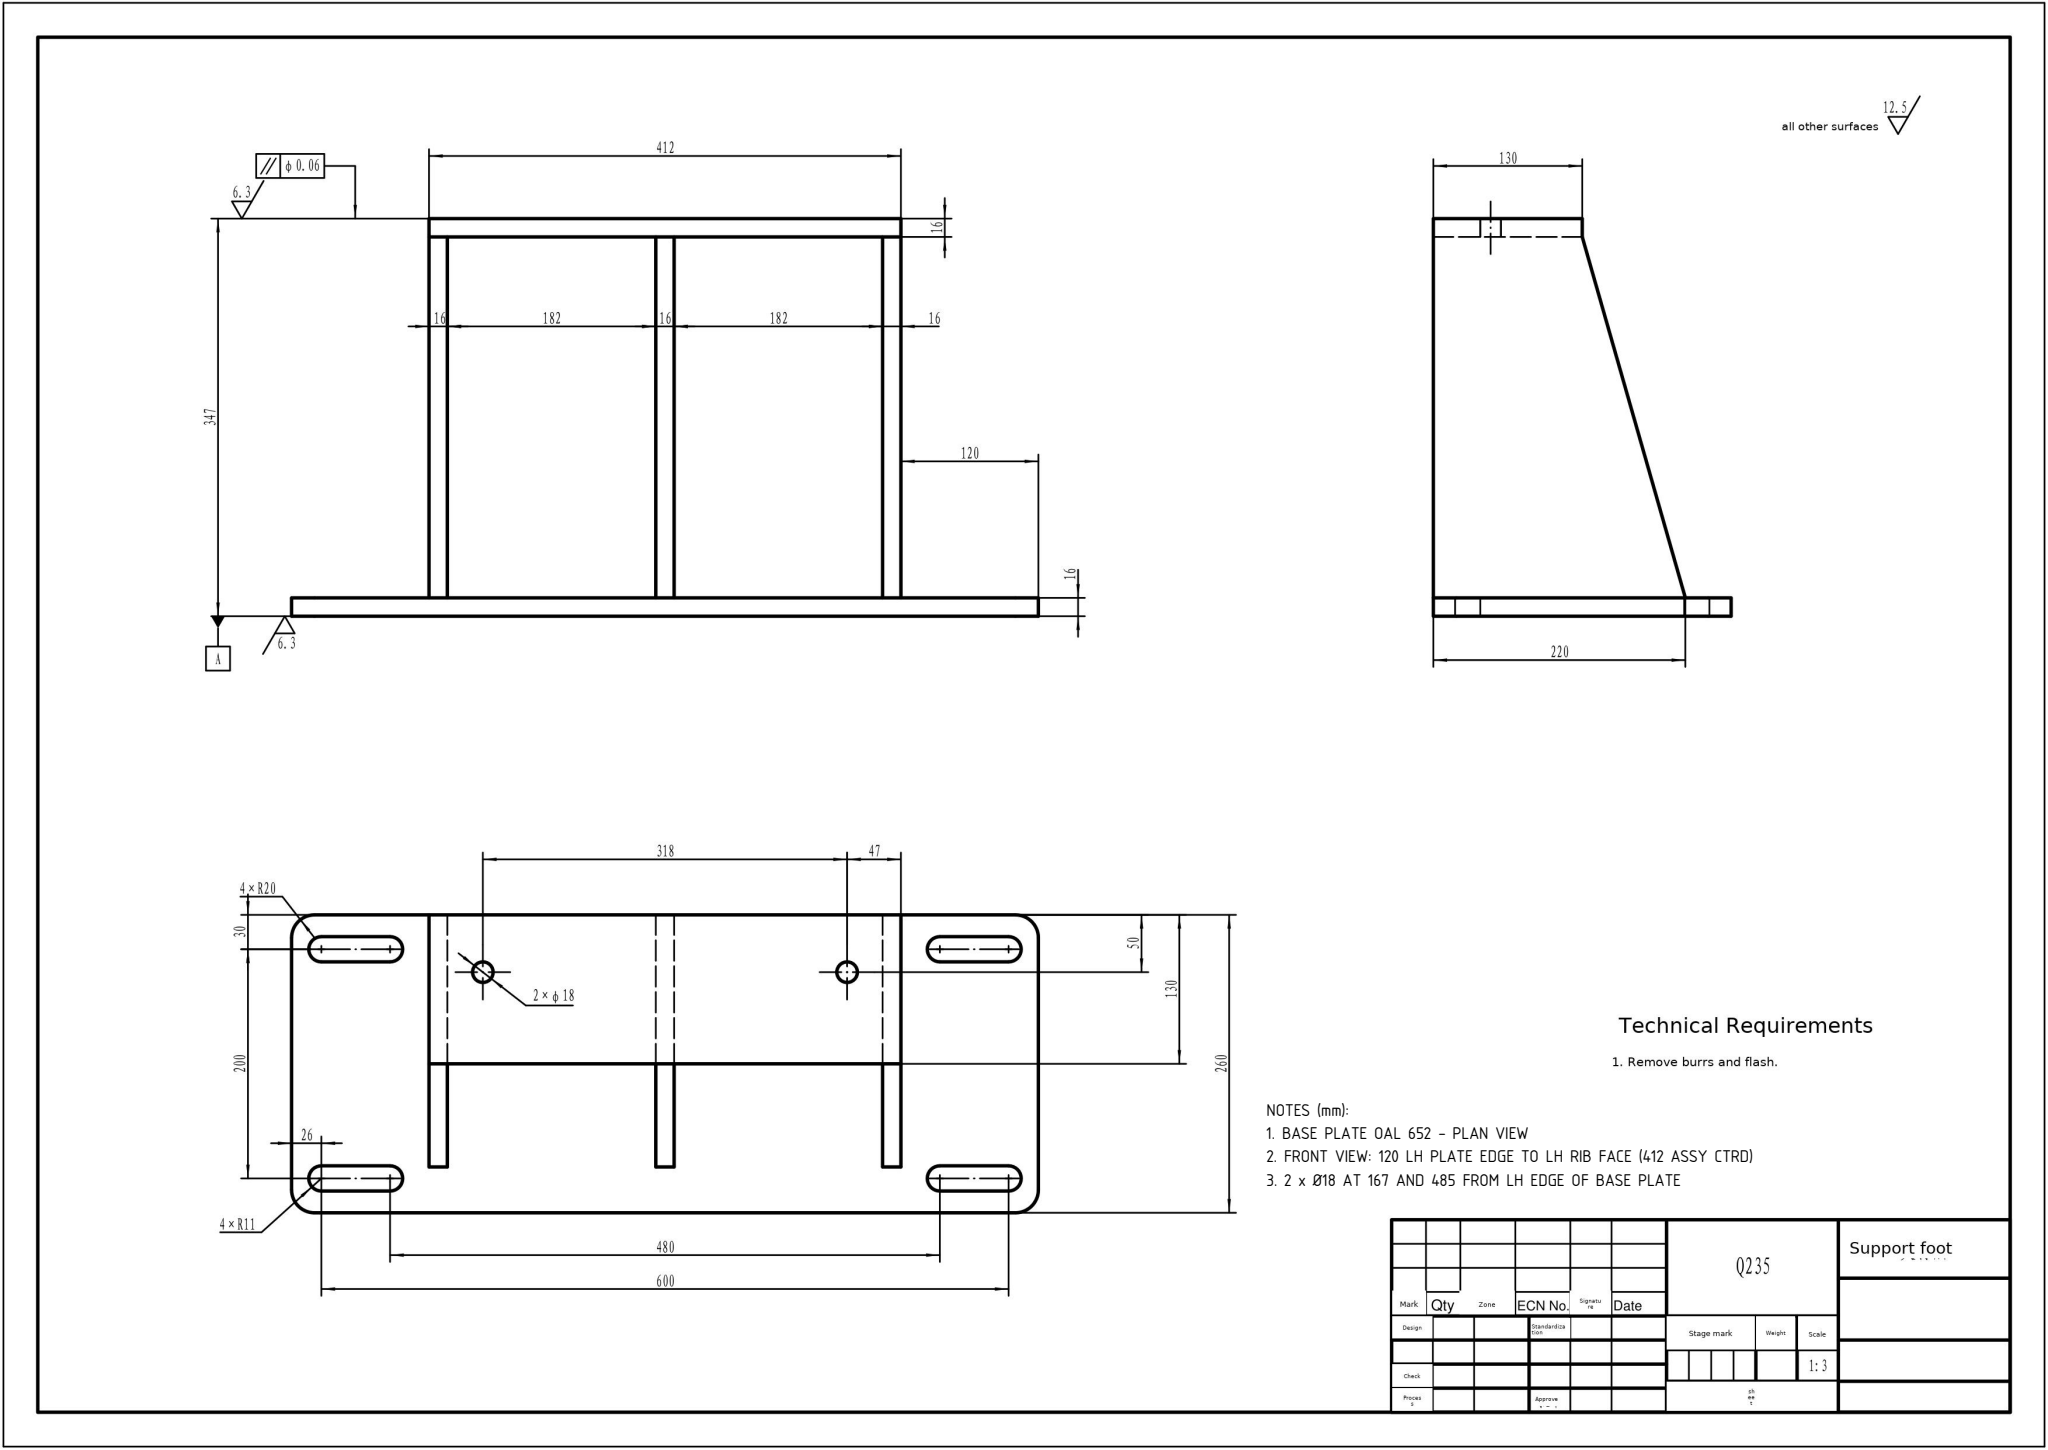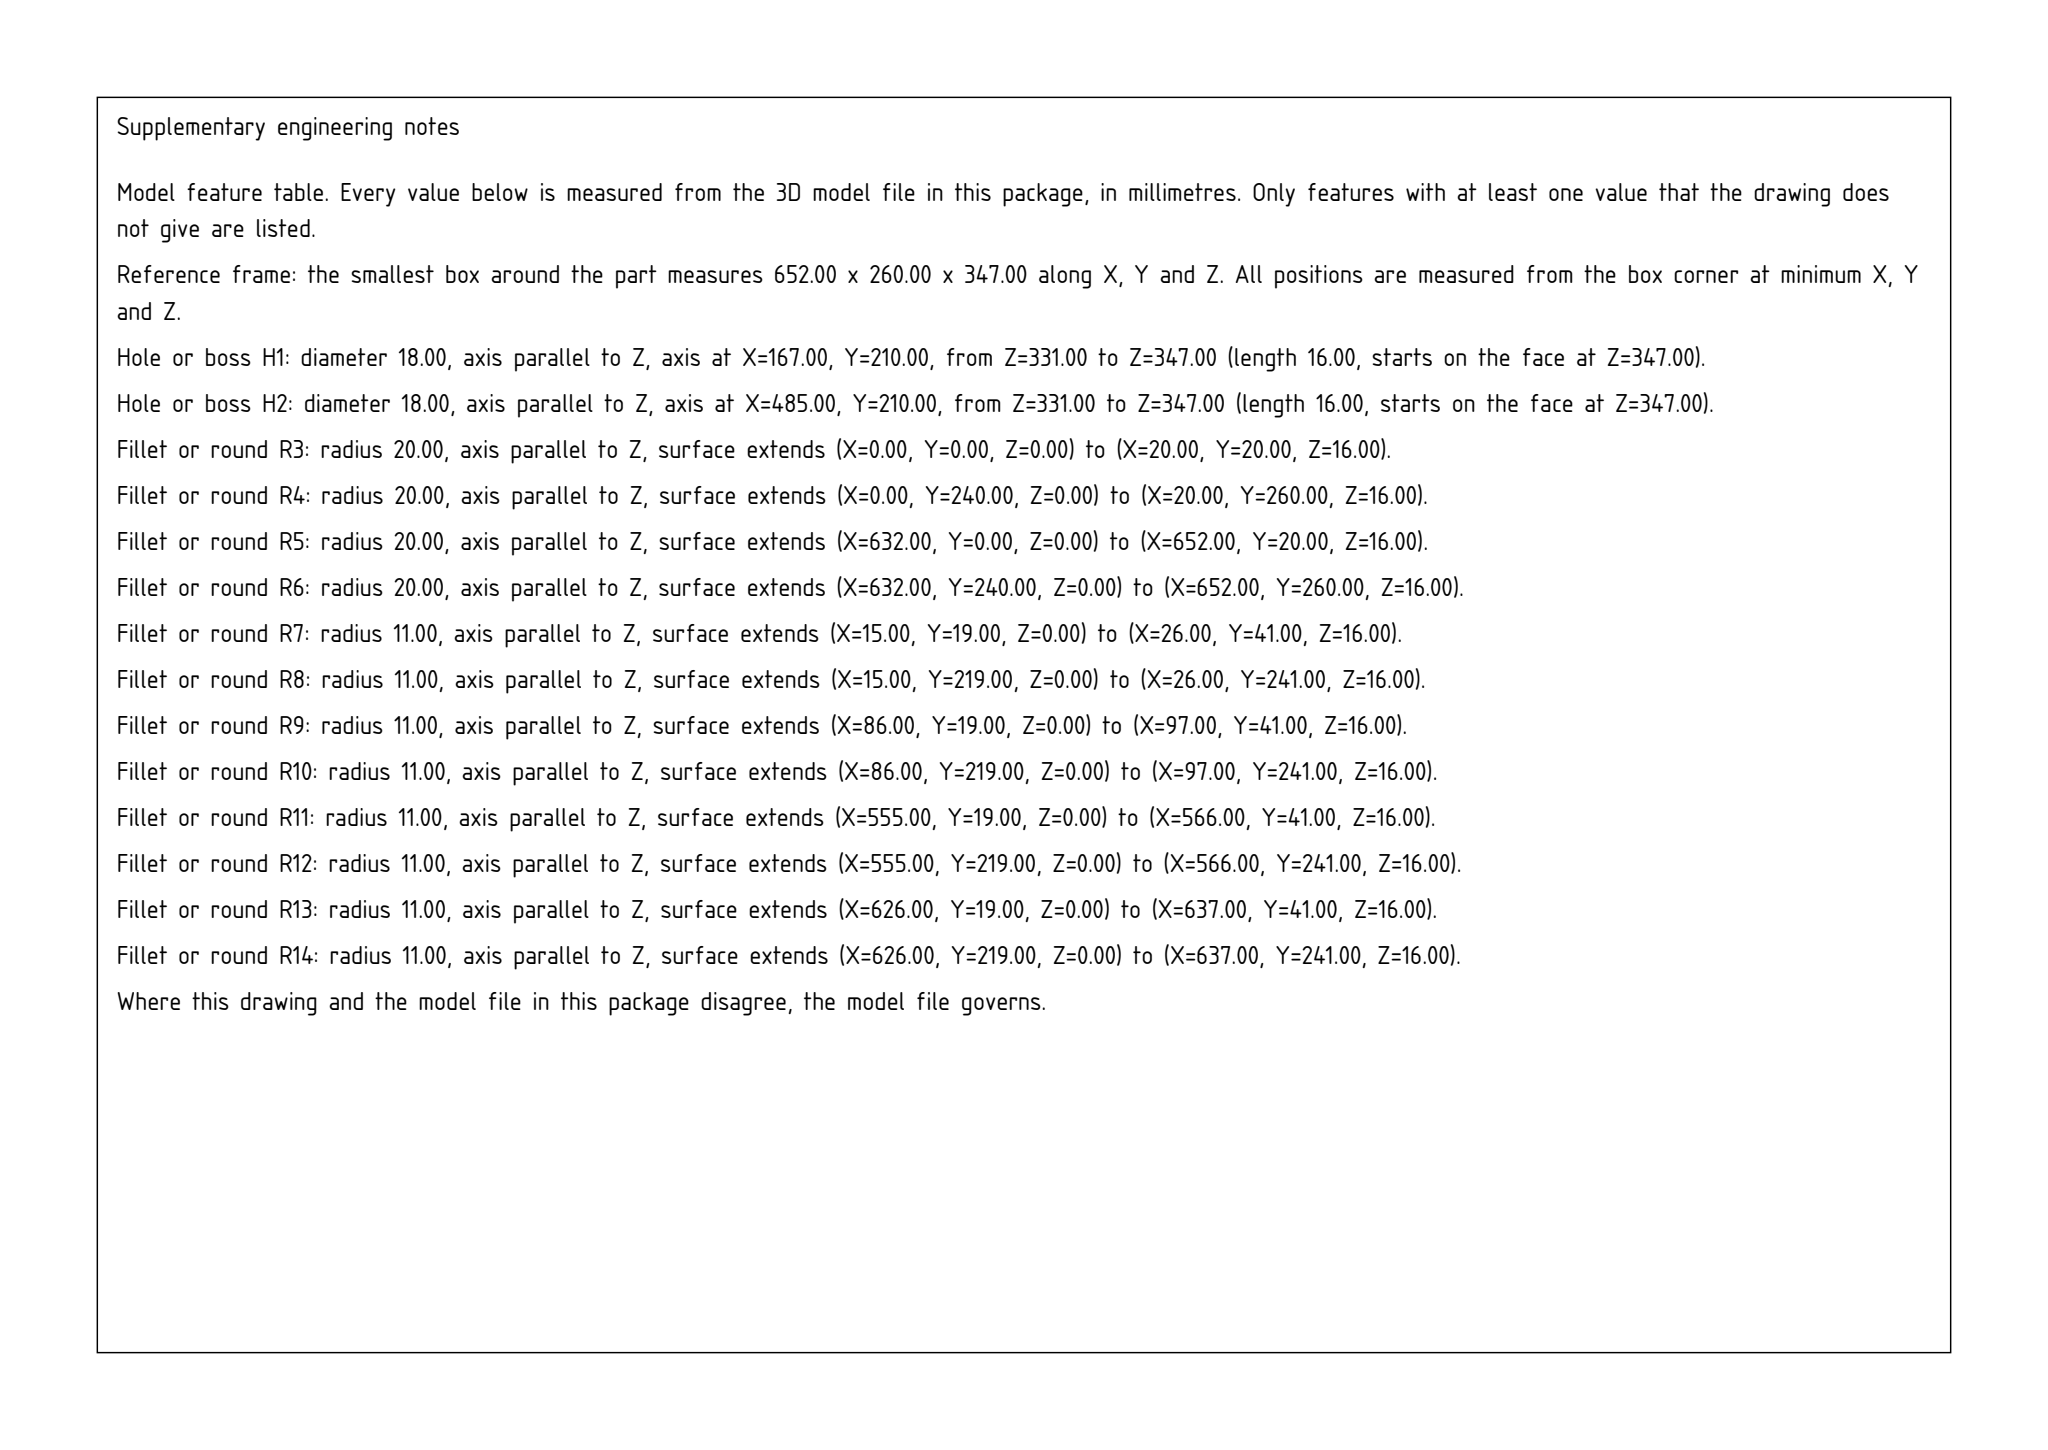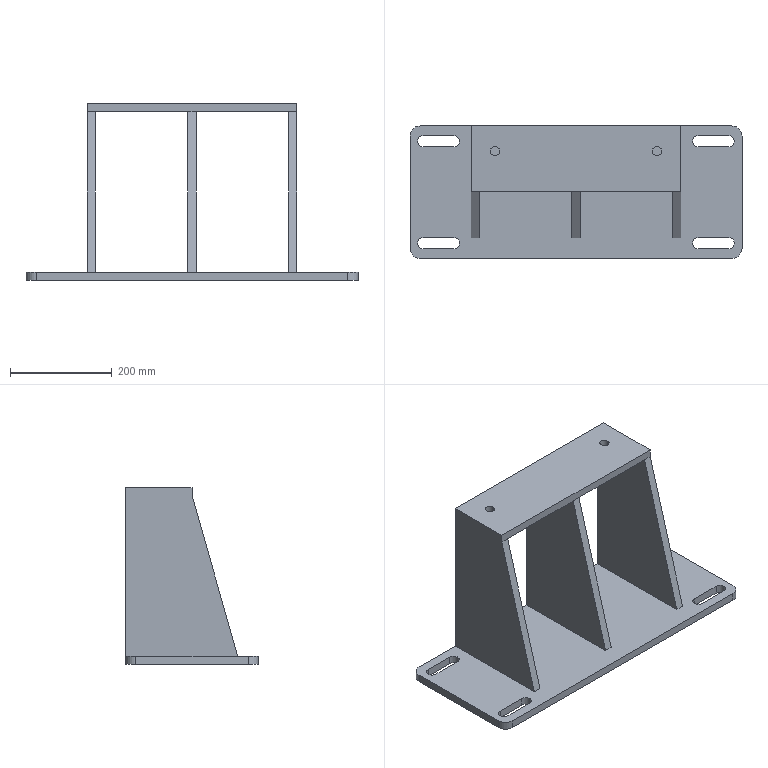Part | SolidWorks | mm | 1 solid | 47 faces | box 652 x 260 x 347 mm | volume 6092835 mm3 | plane 27 | cylinder 20 | commonest cylinder face diameters 22 x12 18 x4 40 x4
Drawing notes:
BASE PLATE OAL 652 - PLAN VIEW | from the solid: bbox_xyz X = 652.0; base plate faces at x=0 and x=652
FRONT VIEW: 120 LH PLATE EDGE TO LH RIB FACE (412 ASSY CTRD) | from the solid: x planes 0, 120, 532, 652; rib/top-plate span 120-532 = 412, symmetric
2 x Ø18 AT 167 AND 485 FROM LH EDGE OF BASE PLATE | from the solid: cylinders dia 18, axis z, pos x=167.0 and x=485.0, y=210
build123d program:
from build123d import *

# Parameters (mm, degrees)
BOSS_EXTRUDE1_DEPTH = 16
BOSS_EXTRUDE2_DEPTH = 16
LPATTERN1_COUNT     = 3
LPATTERN1_PITCH     = 198
SKETCH4_W           = 412
SKETCH4_H           = 130
SKETCH4_R           = 9
BOSS_EXTRUDE4_DEPTH = 16


with BuildPart() as part:
    # Sketch1 → Boss-Extrude1 (new body)
    with BuildSketch(Plane.XY):
        with BuildLine():
            Line((20, 0), (632, 0))
            ThreePointArc((632, 0), (646.142, 5.858), (652, 20))
            Line((652, 20), (652, 240))
            ThreePointArc((652, 240), (646.142, 254.142), (632, 260))
            Line((632, 260), (20, 260))
            ThreePointArc((20, 260), (5.858, 254.142), (0, 240))
            Line((0, 240), (0, 20))
            ThreePointArc((0, 20), (5.858, 5.858), (20, 0))
        make_face()
        with BuildLine():
            Line((26, 241), (86, 241))
            ThreePointArc((86, 241), (97, 230), (86, 219))
            Line((86, 219), (26, 219))
            ThreePointArc((26, 219), (15, 230), (26, 241))
        make_face(mode=Mode.SUBTRACT)
        with BuildLine():
            Line((566, 241), (626, 241))
            ThreePointArc((626, 241), (637, 230), (626, 219))
            Line((626, 219), (566, 219))
            ThreePointArc((566, 219), (555, 230), (566, 241))
        make_face(mode=Mode.SUBTRACT)
        with BuildLine():
            Line((26, 41), (86, 41))
            ThreePointArc((86, 41), (97, 30), (86, 19))
            Line((86, 19), (26, 19))
            ThreePointArc((26, 19), (15, 30), (26, 41))
        make_face(mode=Mode.SUBTRACT)
        with BuildLine():
            Line((566, 41), (626, 41))
            ThreePointArc((626, 41), (637, 30), (626, 19))
            Line((626, 19), (566, 19))
            ThreePointArc((566, 19), (555, 30), (566, 41))
        make_face(mode=Mode.SUBTRACT)
    extrude(amount=BOSS_EXTRUDE1_DEPTH)

    # Sketch2 → Boss-Extrude2 (add)
    with BuildSketch(Plane.ZY.offset(-120)):
        Polygon((331, 260), (331, 130), (16, 40), (16, 260), align=None)
    boss_extrude2 = extrude(amount=-BOSS_EXTRUDE2_DEPTH)

    # LPattern1: Boss-Extrude2 ×3
    with Locations(*[(i * LPATTERN1_PITCH, 0, 0) for i in range(1, LPATTERN1_COUNT)]):
        add(boss_extrude2)


with BuildPart() as body_2:
    # Sketch4 → Boss-Extrude4 (new body)
    with BuildSketch(Plane.XY.offset(331)):
        with Locations((326, 195)):
            Rectangle(SKETCH4_W, SKETCH4_H)
        with Locations((167, 210)):
            Circle(SKETCH4_R, mode=Mode.SUBTRACT)
        with Locations((485, 210)):
            Circle(SKETCH4_R, mode=Mode.SUBTRACT)
    extrude(amount=BOSS_EXTRUDE4_DEPTH)

    # Combine1: union part
    add(part.part)


solid = body_2.part